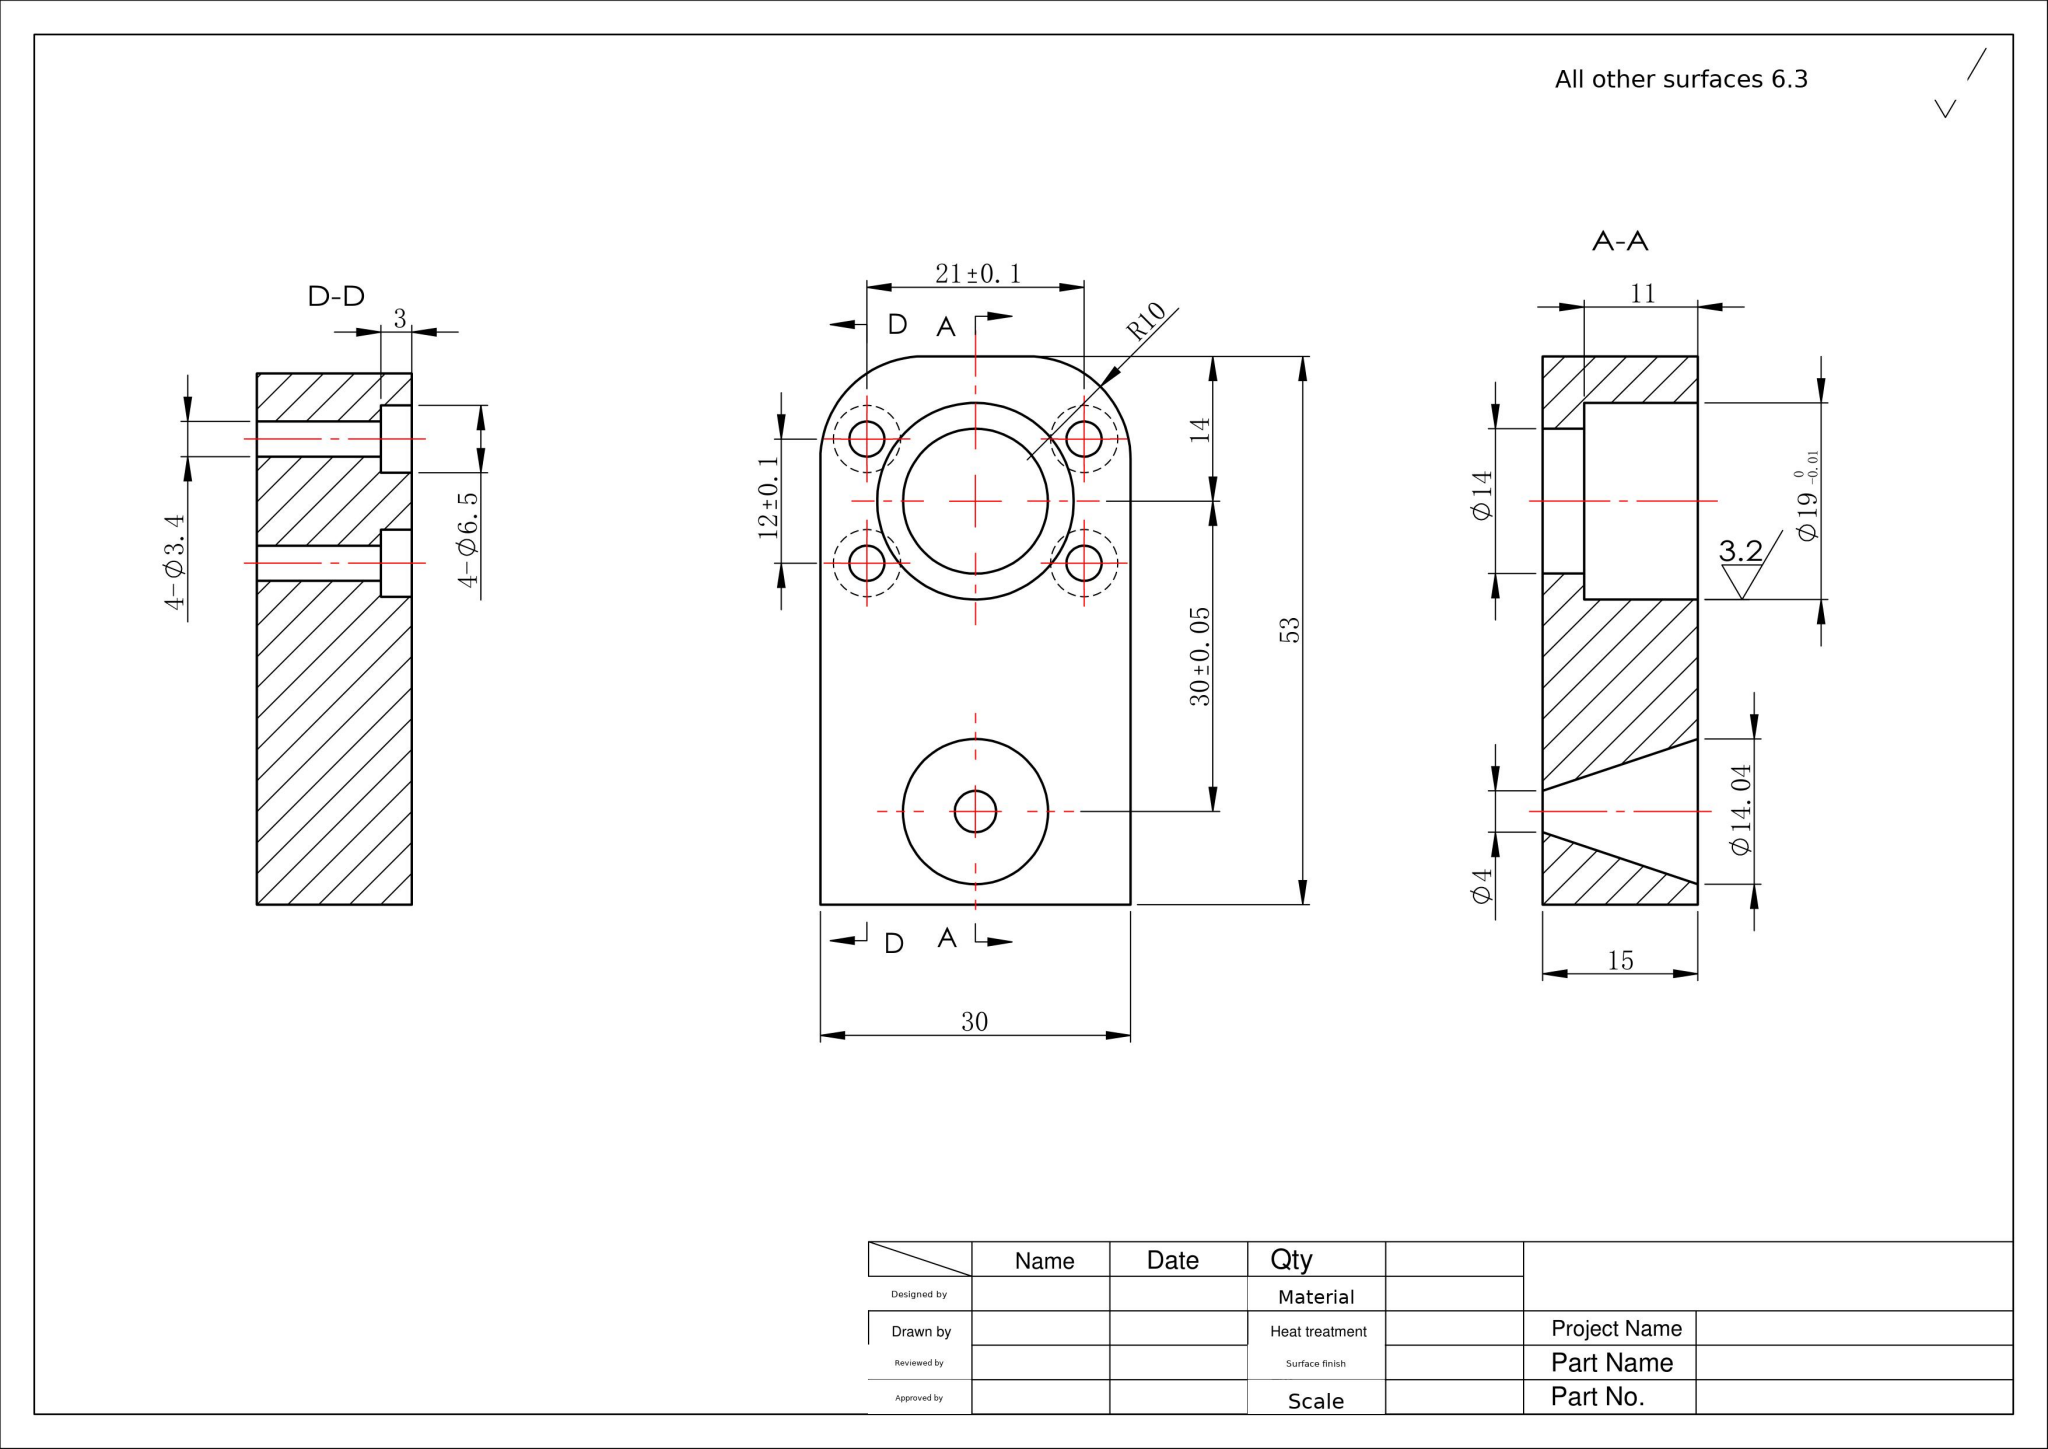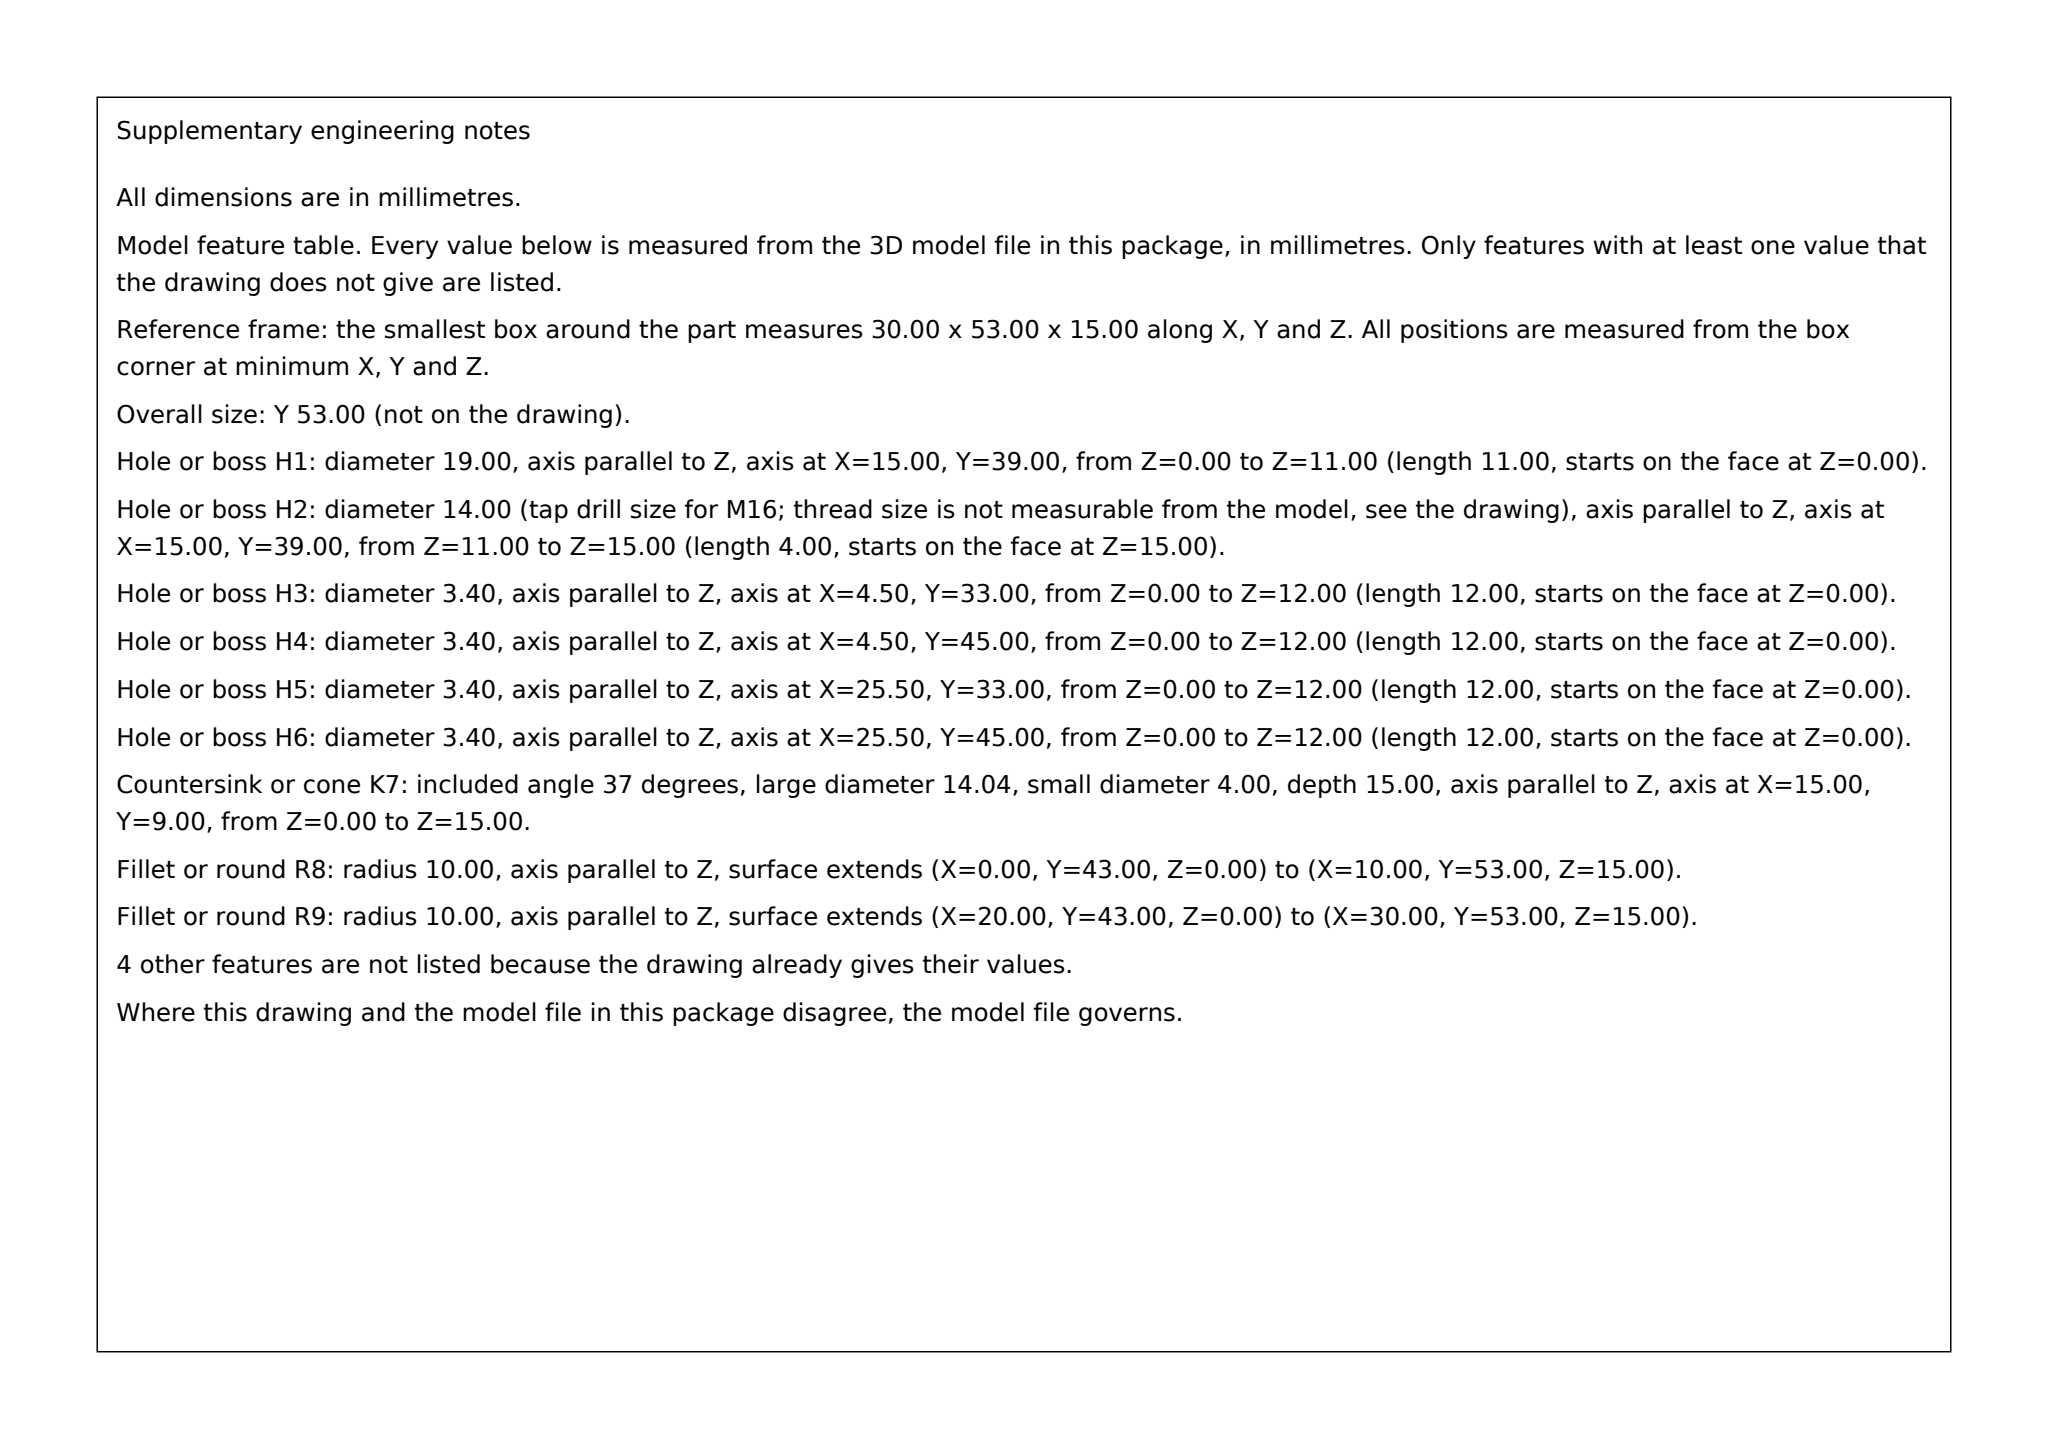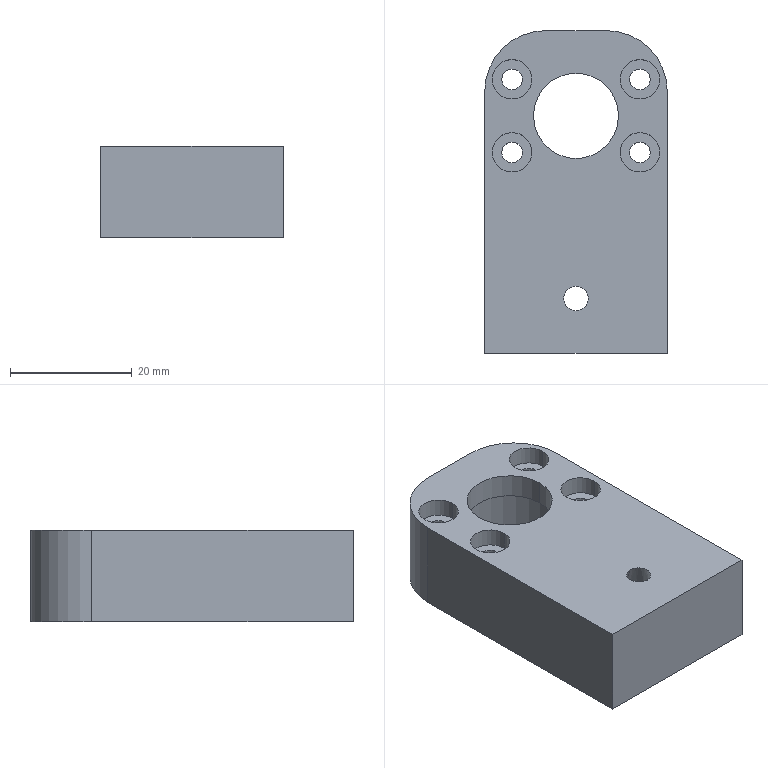Part | SolidWorks | mm | 1 solid | 35 faces | box 30 x 53 x 15 mm | volume 17580 mm3 | cylinder 22 | plane 11 | cone 2 | commonest cylinder face diameters 3.4 x8 6.5 x8 14 x2 19 x2 20 x2
build123d program:
from build123d import *

# Parameters (mm, degrees)
EXTRUDE1_DEPTH     = 15
SKETCH5_R          = 9.5
CUT_EXTRUDE2_DEPTH = 11
SKETCH6_R          = 7
CUT_EXTRUDE3_DEPTH = 62.887
HOLE2_D            = 3.4
HOLE2_CBORE_D      = 6.5
HOLE2_CBORE_DEPTH  = 3


with BuildPart() as part:
    # Sketch1 → Extrude1 (new body)
    with BuildSketch(Plane.XY):
        with BuildLine():
            Line((0, 0), (30, 0))
            Line((30, 0), (30, 43))
            ThreePointArc((30, 43), (27.071, 50.071), (20, 53))
            Line((20, 53), (10, 53))
            ThreePointArc((10, 53), (2.929, 50.071), (0, 43))
            Line((0, 43), (0, 0))
        make_face()
    extrude(amount=EXTRUDE1_DEPTH)

    # Sketch5 → Cut-Extrude2 (cut)
    with BuildSketch(Plane(origin=(0, 0, 0), x_dir=(-1, 0, 0), z_dir=(0, 0, -1))):
        with Locations((-15, 39)):
            Circle(SKETCH5_R)
    extrude(amount=-CUT_EXTRUDE2_DEPTH, mode=Mode.SUBTRACT)

    # Sketch6 → Cut-Extrude3 (cut, through all)
    with BuildSketch(Plane(origin=(0, 0, 11), x_dir=(-1, 0, 0), z_dir=(0, 0, -1))):
        with Locations((-15, 39)):
            Circle(SKETCH6_R)
    extrude(amount=-CUT_EXTRUDE3_DEPTH, mode=Mode.SUBTRACT)

    # Hole2 (through all)
    with Locations(Plane(origin=(4.5, 45, 15), x_dir=(1, 0, 0), z_dir=(0, 0, 1))):
        with Locations((0, 0), (0, -12), (21, 0), (21, -12)):
            CounterBoreHole(HOLE2_D / 2, HOLE2_CBORE_D / 2, HOLE2_CBORE_DEPTH)

    # Sketch18 → Cut-Revolve1 (revolve, cut)
    with BuildSketch(Plane(origin=(15, 0, 0), x_dir=(0, 0, -1), z_dir=(1, 0, 0))):
        Polygon((0, 16.019), (-15, 11), (-15, 9), (0, 9), align=None)
    revolve(axis=Axis((15, 9, 15), (0, 0, -1)), mode=Mode.SUBTRACT)


solid = part.part